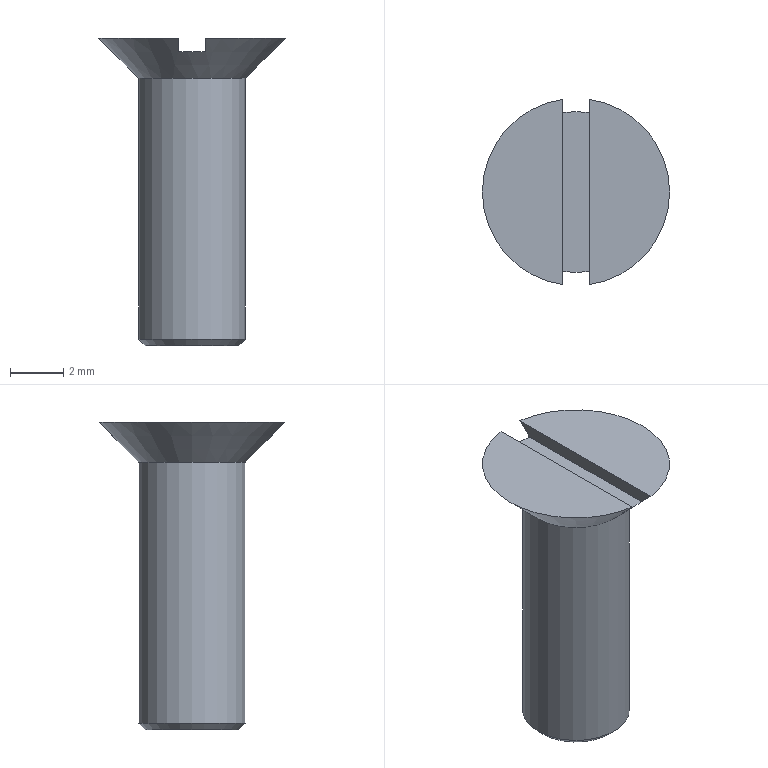Component | NX | FIXING_SCREW_3 | 1 solid | 9 faces | volume 159 mm3 | plane 6 | cone 2 | cylinder 1 | commonest cylinder face diameters 4 x1